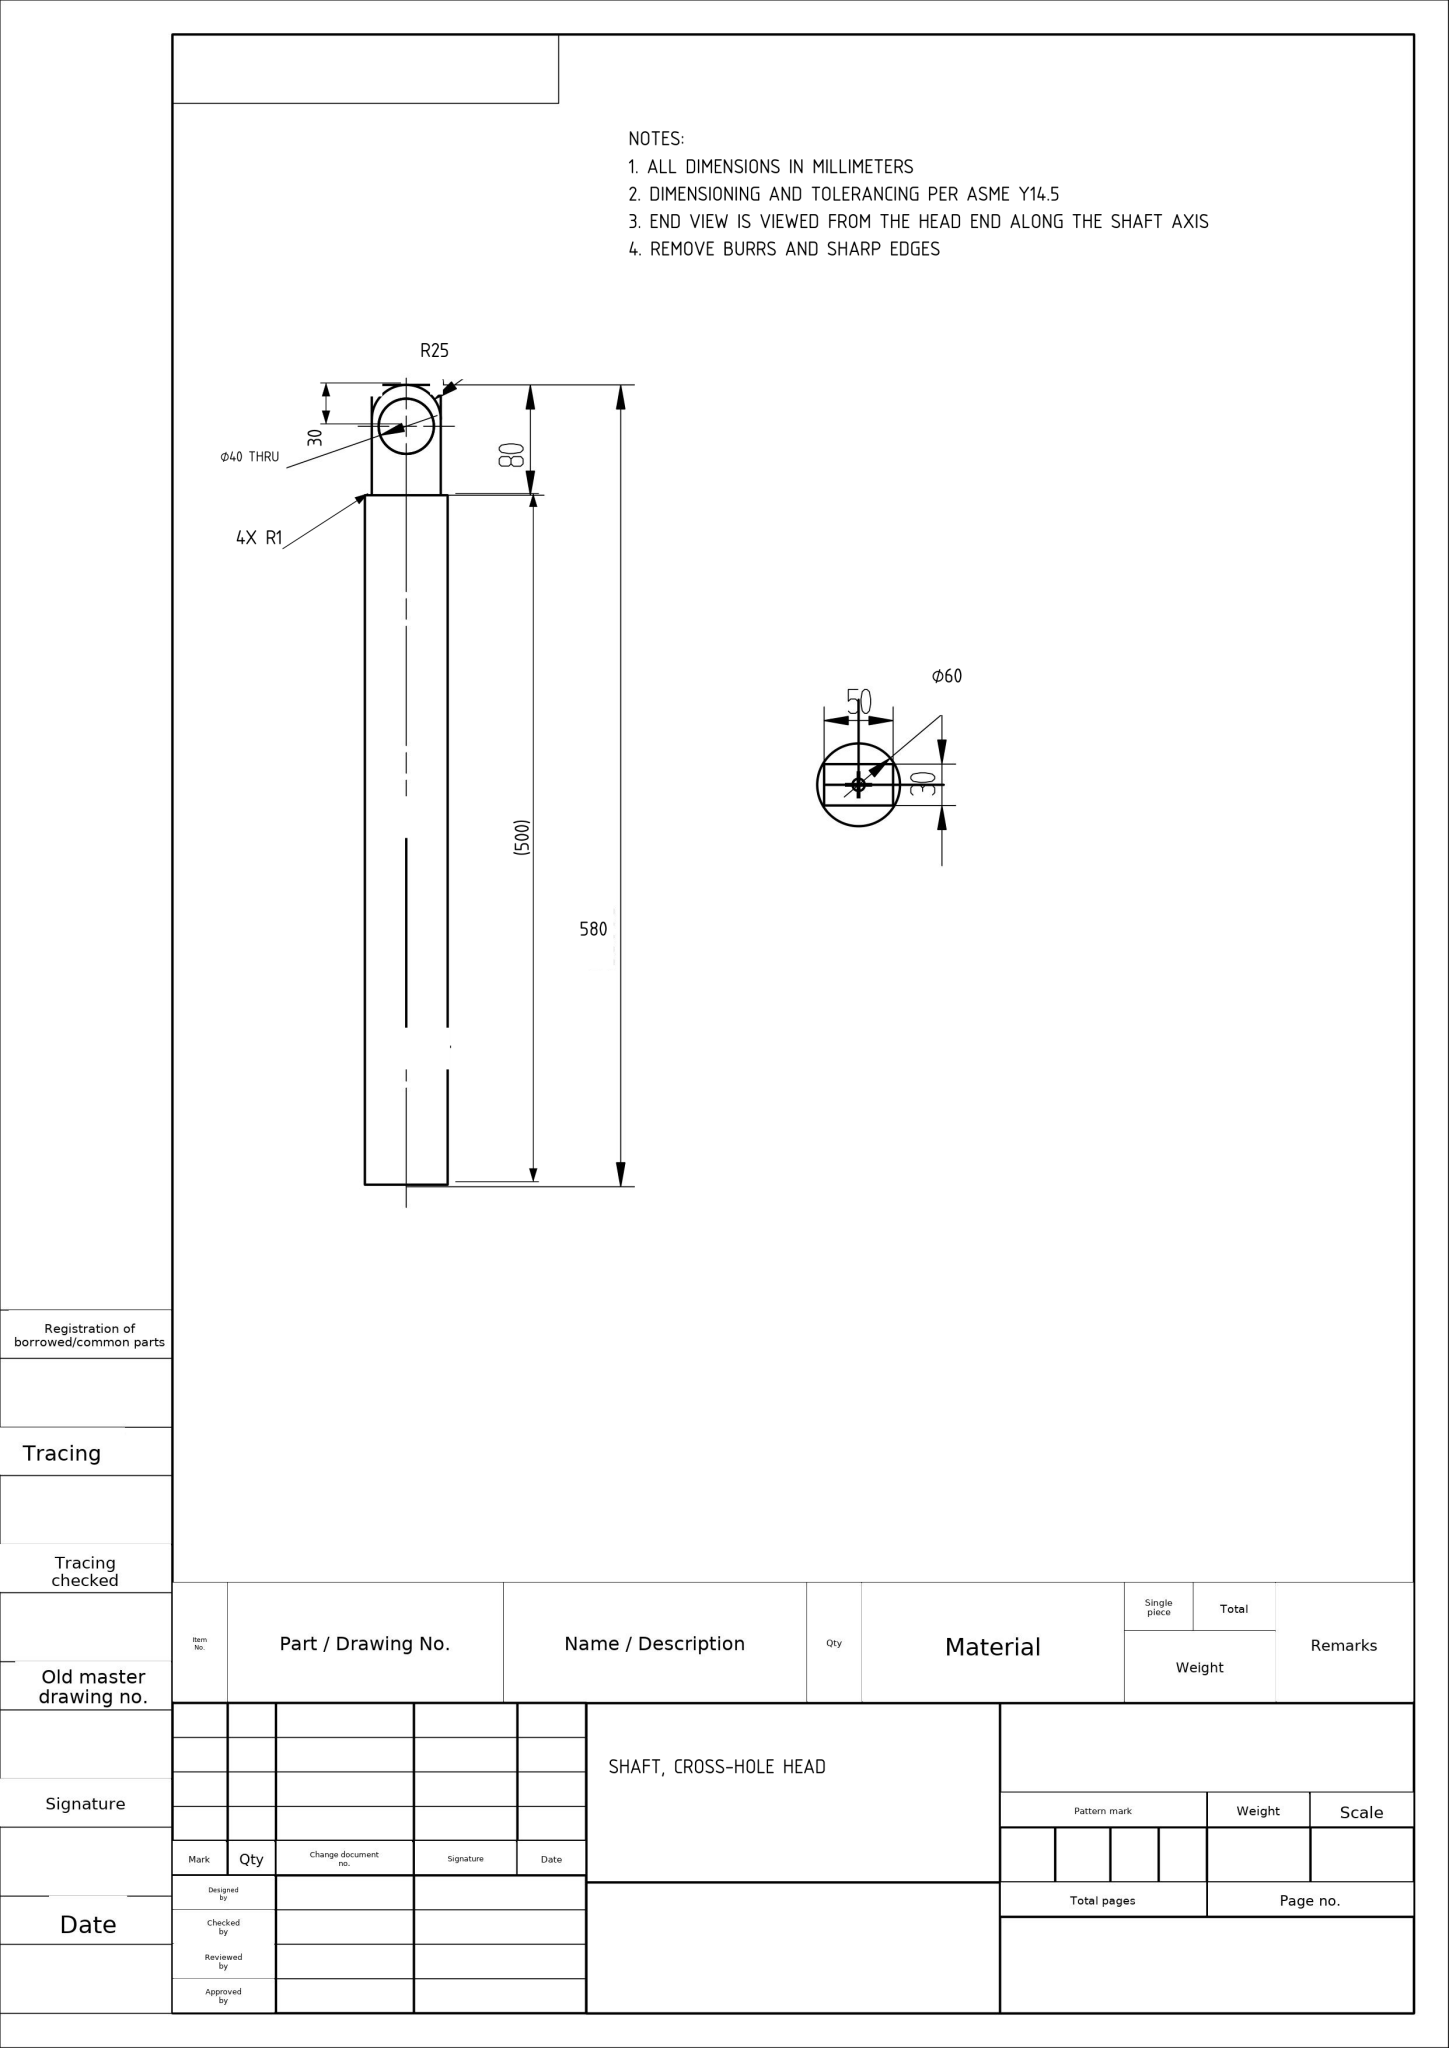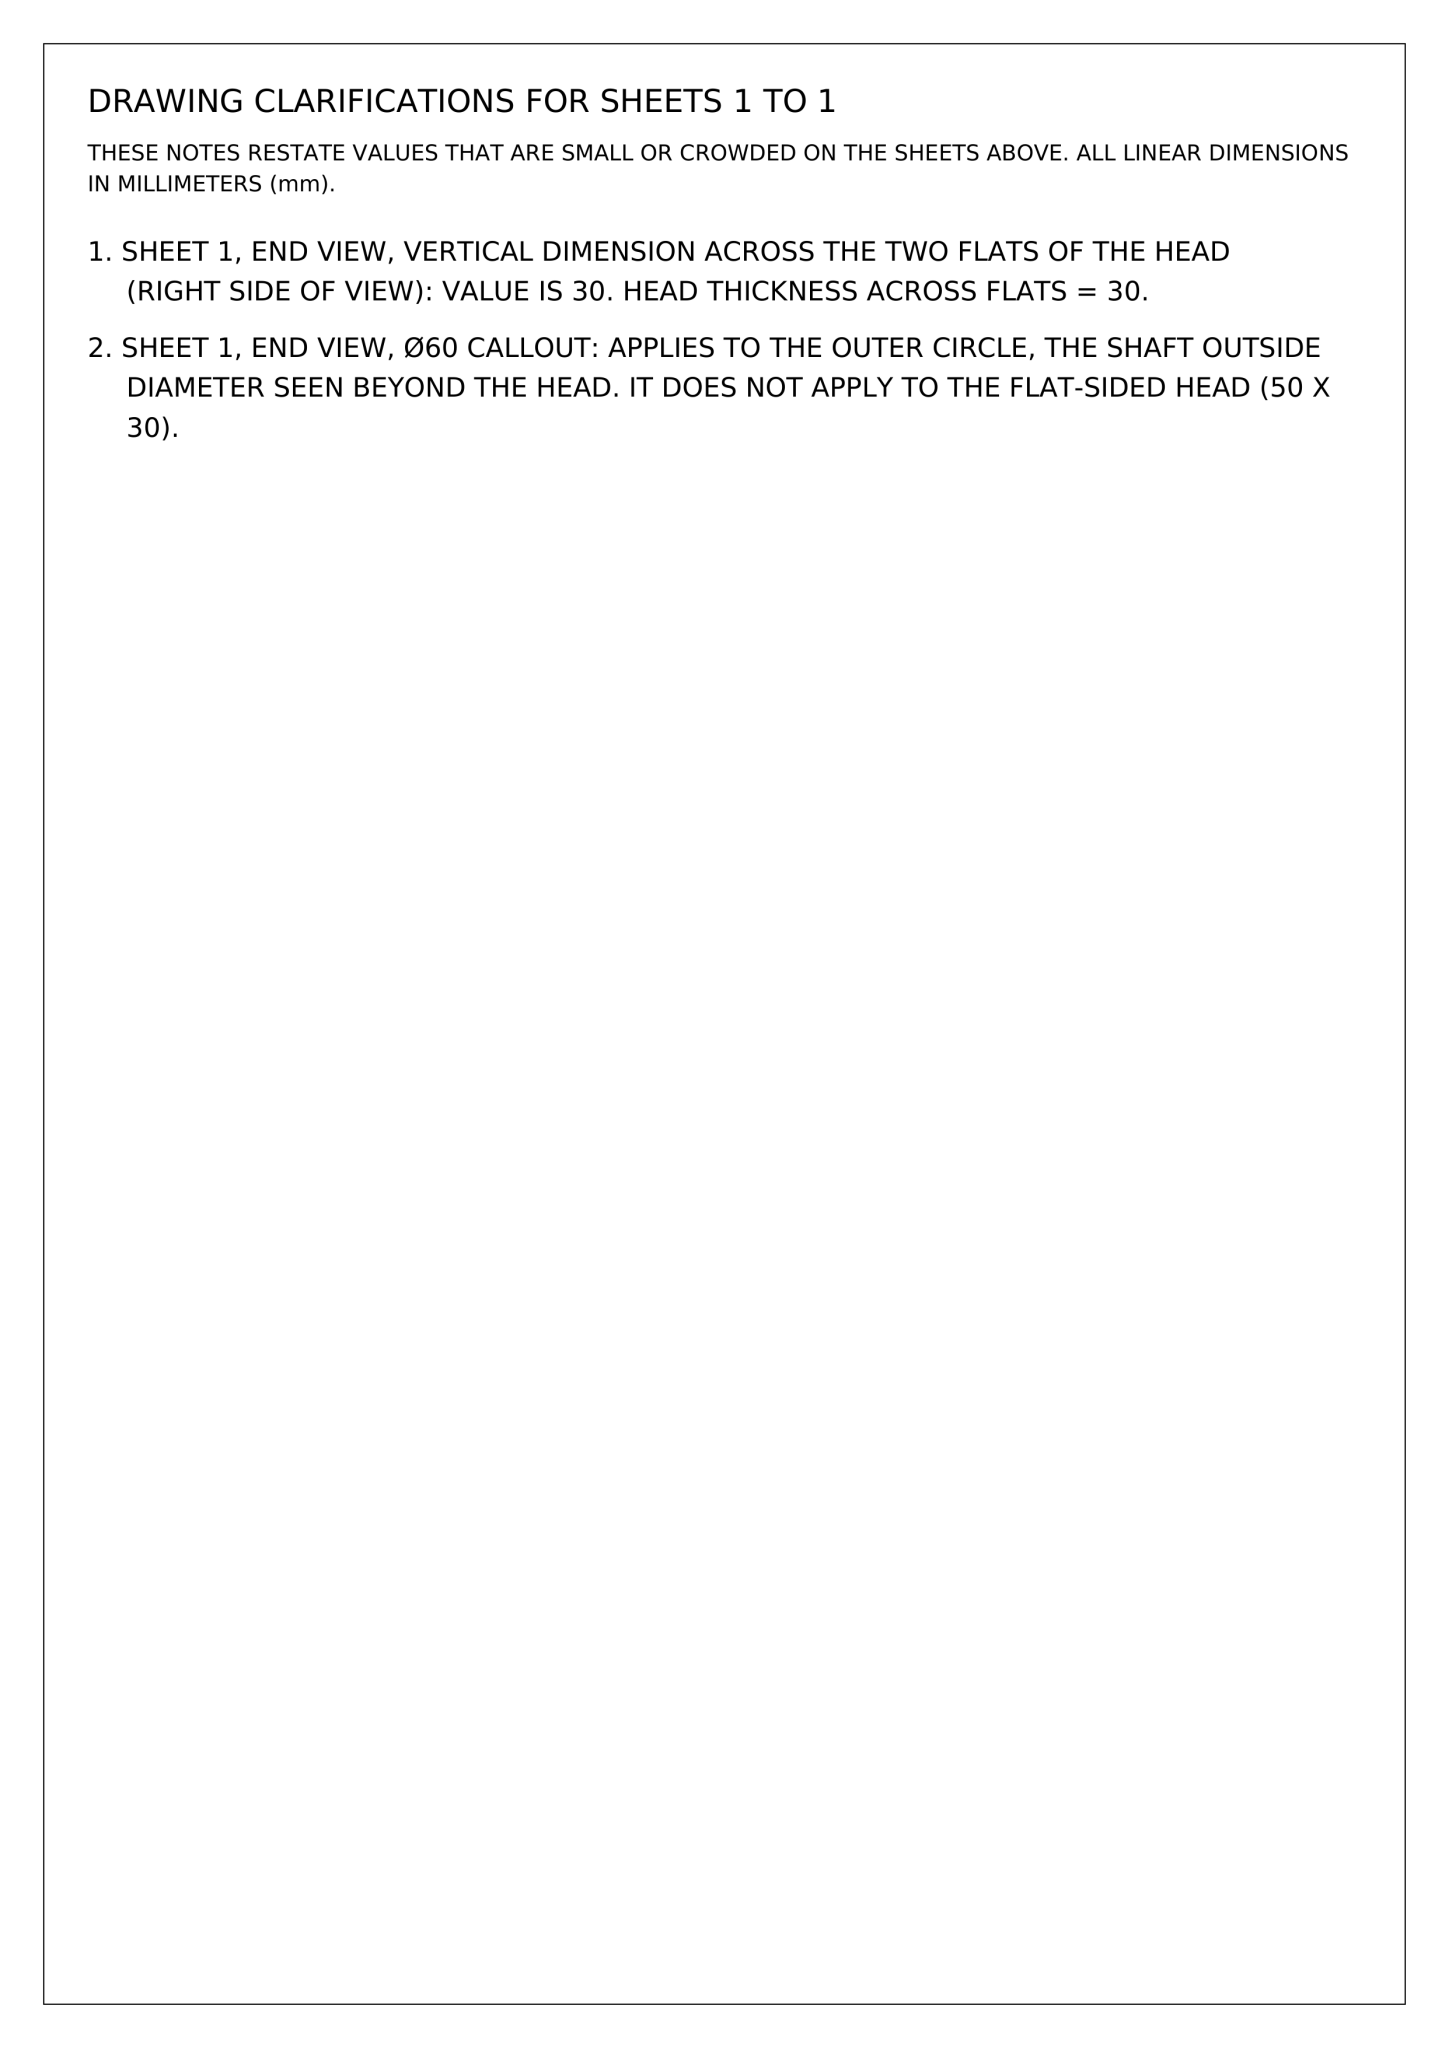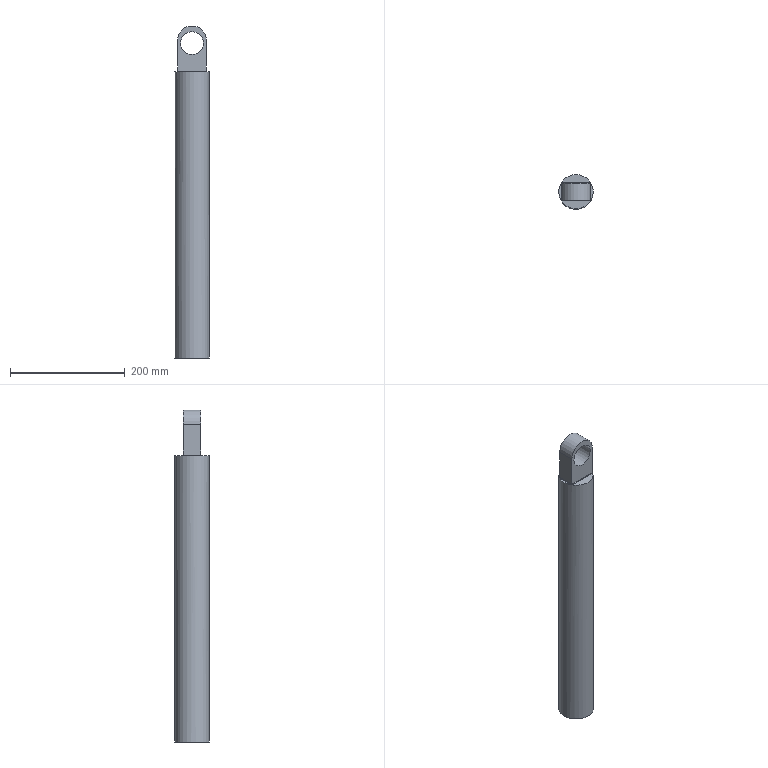Part | NX | mm | 1 solid | 18 faces | box 60 x 60 x 580 mm | volume 1488005 mm3 | plane 9 | cylinder 7 | spline 2 | commonest cylinder face diameters 2 x4 60 x1 40 x1 50 x1
STEP:
#1=CARTESIAN_POINT('',(0.,0.,0.));
#2=DIRECTION('',(0.,0.,1.));
#3=DIRECTION('',(1.,0.,0.));
#4=AXIS2_PLACEMENT_3D('',#1,#2,#3);
#5=(LENGTH_UNIT()NAMED_UNIT(*)SI_UNIT(.MILLI.,.METRE.));
#6=UNCERTAINTY_MEASURE_WITH_UNIT(LENGTH_MEASURE(0.0508),#5,'','');
#7=(NAMED_UNIT(*)PLANE_ANGLE_UNIT()SI_UNIT($,.RADIAN.));
#8=PLANE_ANGLE_MEASURE_WITH_UNIT(PLANE_ANGLE_MEASURE(0.01745),#7);
#9=DIMENSIONAL_EXPONENTS(0.,0.,0.,0.,0.,0.,0.);
#10=(CONVERSION_BASED_UNIT('',#8)NAMED_UNIT(#9)PLANE_ANGLE_UNIT());
#11=(NAMED_UNIT(*)SI_UNIT($,.STERADIAN.)SOLID_ANGLE_UNIT());
#12=(GEOMETRIC_REPRESENTATION_CONTEXT(3)GLOBAL_UNCERTAINTY_ASSIGNED_CONTEXT((#6))GLOBAL_UNIT_ASSIGNED_CONTEXT((#5,#10,#11))REPRESENTATION_CONTEXT('',''));
#13=SHAPE_REPRESENTATION('',(#4),#12);
#14=CARTESIAN_POINT('',(25.377,16.,400.));
#15=VERTEX_POINT('',#14);
#16=CARTESIAN_POINT('',(-25.377,16.,400.));
#17=VERTEX_POINT('',#16);
#18=CARTESIAN_POINT('',(0.,0.,400.));
#19=DIRECTION('',(0.,0.,1.));
#20=DIRECTION('',(1.,0.,0.));
#21=AXIS2_PLACEMENT_3D('',#18,#19,#20);
#22=CIRCLE('',#21,30.);
#23=EDGE_CURVE('',#15,#17,#22,.T.);
#24=ORIENTED_EDGE('',*,*,#23,.T.);
#25=CARTESIAN_POINT('',(0.,16.,400.));
#26=DIRECTION('',(1.,0.,0.));
#27=VECTOR('',#26,1.);
#28=LINE('',#25,#27);
#29=EDGE_CURVE('',#17,#15,#28,.T.);
#30=ORIENTED_EDGE('',*,*,#29,.T.);
#31=EDGE_LOOP('',(#24,#30));
#32=FACE_OUTER_BOUND('',#31,.T.);
#33=CARTESIAN_POINT('',(0.,0.,400.));
#34=DIRECTION('',(0.,0.,1.));
#35=DIRECTION('',(1.,0.,0.));
#36=AXIS2_PLACEMENT_3D('',#33,#34,#35);
#37=PLANE('',#36);
#38=ADVANCED_FACE('',(#32),#37,.T.);
#39=CARTESIAN_POINT('',(-26.,14.967,400.));
#40=VERTEX_POINT('',#39);
#41=CARTESIAN_POINT('',(-26.,-14.967,400.));
#42=VERTEX_POINT('',#41);
#43=CARTESIAN_POINT('',(0.,0.,400.));
#44=DIRECTION('',(0.,0.,1.));
#45=DIRECTION('',(1.,0.,0.));
#46=AXIS2_PLACEMENT_3D('',#43,#44,#45);
#47=CIRCLE('',#46,30.);
#48=EDGE_CURVE('',#40,#42,#47,.T.);
#49=ORIENTED_EDGE('',*,*,#48,.T.);
#50=CARTESIAN_POINT('',(-26.,0.,400.));
#51=DIRECTION('',(0.,1.,0.));
#52=VECTOR('',#51,1.);
#53=LINE('',#50,#52);
#54=EDGE_CURVE('',#42,#40,#53,.T.);
#55=ORIENTED_EDGE('',*,*,#54,.T.);
#56=EDGE_LOOP('',(#49,#55));
#57=FACE_OUTER_BOUND('',#56,.T.);
#58=CARTESIAN_POINT('',(0.,0.,400.));
#59=DIRECTION('',(0.,0.,1.));
#60=DIRECTION('',(1.,0.,0.));
#61=AXIS2_PLACEMENT_3D('',#58,#59,#60);
#62=PLANE('',#61);
#63=ADVANCED_FACE('',(#57),#62,.T.);
#64=CARTESIAN_POINT('',(26.,-14.967,400.));
#65=VERTEX_POINT('',#64);
#66=CARTESIAN_POINT('',(26.,14.967,400.));
#67=VERTEX_POINT('',#66);
#68=CARTESIAN_POINT('',(0.,0.,400.));
#69=DIRECTION('',(0.,0.,1.));
#70=DIRECTION('',(1.,0.,0.));
#71=AXIS2_PLACEMENT_3D('',#68,#69,#70);
#72=CIRCLE('',#71,30.);
#73=EDGE_CURVE('',#65,#67,#72,.T.);
#74=ORIENTED_EDGE('',*,*,#73,.T.);
#75=CARTESIAN_POINT('',(26.,0.,400.));
#76=DIRECTION('',(0.,-1.,0.));
#77=VECTOR('',#76,1.);
#78=LINE('',#75,#77);
#79=EDGE_CURVE('',#67,#65,#78,.T.);
#80=ORIENTED_EDGE('',*,*,#79,.T.);
#81=EDGE_LOOP('',(#74,#80));
#82=FACE_OUTER_BOUND('',#81,.T.);
#83=CARTESIAN_POINT('',(0.,0.,400.));
#84=DIRECTION('',(0.,0.,1.));
#85=DIRECTION('',(1.,0.,0.));
#86=AXIS2_PLACEMENT_3D('',#83,#84,#85);
#87=PLANE('',#86);
#88=ADVANCED_FACE('',(#82),#87,.T.);
#89=CARTESIAN_POINT('',(-25.377,-16.,400.));
#90=VERTEX_POINT('',#89);
#91=CARTESIAN_POINT('',(25.377,-16.,400.));
#92=VERTEX_POINT('',#91);
#93=CARTESIAN_POINT('',(0.,0.,400.));
#94=DIRECTION('',(0.,0.,1.));
#95=DIRECTION('',(1.,0.,0.));
#96=AXIS2_PLACEMENT_3D('',#93,#94,#95);
#97=CIRCLE('',#96,30.);
#98=EDGE_CURVE('',#90,#92,#97,.T.);
#99=ORIENTED_EDGE('',*,*,#98,.T.);
#100=CARTESIAN_POINT('',(-25.,-16.,400.));
#101=DIRECTION('',(-1.,0.,0.));
#102=VECTOR('',#101,1.);
#103=LINE('',#100,#102);
#104=EDGE_CURVE('',#92,#90,#103,.T.);
#105=ORIENTED_EDGE('',*,*,#104,.T.);
#106=EDGE_LOOP('',(#99,#105));
#107=FACE_OUTER_BOUND('',#106,.T.);
#108=CARTESIAN_POINT('',(0.,0.,400.));
#109=DIRECTION('',(0.,0.,1.));
#110=DIRECTION('',(1.,0.,0.));
#111=AXIS2_PLACEMENT_3D('',#108,#109,#110);
#112=PLANE('',#111);
#113=ADVANCED_FACE('',(#107),#112,.T.);
#114=CARTESIAN_POINT('',(25.616,15.616,400.077));
#115=VERTEX_POINT('',#114);
#116=CARTESIAN_POINT('',(25.377,16.,400.));
#117=CARTESIAN_POINT('',(25.459,15.871,400.));
#118=CARTESIAN_POINT('',(25.541,15.739,400.026));
#119=CARTESIAN_POINT('',(25.616,15.616,400.077));
#120=B_SPLINE_CURVE_WITH_KNOTS('',3,(#116,#117,#118,#119),.UNSPECIFIED.,.F.,.F.,(4,4),(0.,1.),.UNSPECIFIED.);
#121=EDGE_CURVE('',#15,#115,#120,.T.);
#122=ORIENTED_EDGE('',*,*,#121,.T.);
#123=CARTESIAN_POINT('',(26.,14.967,400.));
#124=CARTESIAN_POINT('',(25.874,15.186,400.));
#125=CARTESIAN_POINT('',(25.744,15.405,400.023));
#126=CARTESIAN_POINT('',(25.616,15.616,400.077));
#127=B_SPLINE_CURVE_WITH_KNOTS('',3,(#123,#124,#125,#126),.UNSPECIFIED.,.F.,.F.,(4,4),(0.,1.),.UNSPECIFIED.);
#128=EDGE_CURVE('',#67,#115,#127,.T.);
#129=ORIENTED_EDGE('',*,*,#128,.F.);
#130=ORIENTED_EDGE('',*,*,#73,.F.);
#131=CARTESIAN_POINT('',(25.377,-16.,400.));
#132=CARTESIAN_POINT('',(25.379,-15.998,400.));
#133=CARTESIAN_POINT('',(25.38,-15.996,400.));
#134=CARTESIAN_POINT('',(25.419,-15.934,400.));
#135=CARTESIAN_POINT('',(25.458,-15.871,400.));
#136=CARTESIAN_POINT('',(25.539,-15.741,400.));
#137=CARTESIAN_POINT('',(25.58,-15.674,400.));
#138=CARTESIAN_POINT('',(25.663,-15.538,400.));
#139=CARTESIAN_POINT('',(25.705,-15.469,400.));
#140=CARTESIAN_POINT('',(25.83,-15.259,400.));
#141=CARTESIAN_POINT('',(25.915,-15.114,400.));
#142=CARTESIAN_POINT('',(26.,-14.967,400.));
#143=(BOUNDED_CURVE()B_SPLINE_CURVE(3,(#131,#132,#133,#134,#135,#136,#137,#138,#139,#140,#141,#142),.UNSPECIFIED.,.F.,.F.)B_SPLINE_CURVE_WITH_KNOTS((4,2,2,2,2,4),(0.,0.00739,0.2059,0.4044,0.603,1.),.UNSPECIFIED.)CURVE()GEOMETRIC_REPRESENTATION_ITEM()RATIONAL_B_SPLINE_CURVE((1.,1.,1.,1.,1.,1.,1.,1.,1.,1.,1.,1.))REPRESENTATION_ITEM(''));
#144=EDGE_CURVE('',#92,#65,#143,.T.);
#145=ORIENTED_EDGE('',*,*,#144,.F.);
#146=ORIENTED_EDGE('',*,*,#98,.F.);
#147=CARTESIAN_POINT('',(-26.,-14.967,400.));
#148=CARTESIAN_POINT('',(-25.915,-15.114,400.));
#149=CARTESIAN_POINT('',(-25.83,-15.259,400.));
#150=CARTESIAN_POINT('',(-25.705,-15.469,400.));
#151=CARTESIAN_POINT('',(-25.663,-15.538,400.));
#152=CARTESIAN_POINT('',(-25.58,-15.674,400.));
#153=CARTESIAN_POINT('',(-25.539,-15.741,400.));
#154=CARTESIAN_POINT('',(-25.458,-15.871,400.));
#155=CARTESIAN_POINT('',(-25.419,-15.934,400.));
#156=CARTESIAN_POINT('',(-25.38,-15.996,400.));
#157=CARTESIAN_POINT('',(-25.379,-15.998,400.));
#158=CARTESIAN_POINT('',(-25.377,-16.,400.));
#159=(BOUNDED_CURVE()B_SPLINE_CURVE(3,(#147,#148,#149,#150,#151,#152,#153,#154,#155,#156,#157,#158),.UNSPECIFIED.,.F.,.F.)B_SPLINE_CURVE_WITH_KNOTS((4,2,2,2,2,4),(0.,0.397,0.5956,0.7941,0.9926,1.),.UNSPECIFIED.)CURVE()GEOMETRIC_REPRESENTATION_ITEM()RATIONAL_B_SPLINE_CURVE((1.,1.,1.,1.,1.,1.,1.,1.,1.,1.,1.,1.))REPRESENTATION_ITEM(''));
#160=EDGE_CURVE('',#42,#90,#159,.T.);
#161=ORIENTED_EDGE('',*,*,#160,.F.);
#162=ORIENTED_EDGE('',*,*,#48,.F.);
#163=CARTESIAN_POINT('',(-25.616,15.616,400.077));
#164=VERTEX_POINT('',#163);
#165=CARTESIAN_POINT('',(-25.616,15.616,400.077));
#166=CARTESIAN_POINT('',(-25.744,15.405,400.023));
#167=CARTESIAN_POINT('',(-25.874,15.186,400.));
#168=CARTESIAN_POINT('',(-26.,14.967,400.));
#169=B_SPLINE_CURVE_WITH_KNOTS('',3,(#165,#166,#167,#168),.UNSPECIFIED.,.F.,.F.,(4,4),(0.,1.),.UNSPECIFIED.);
#170=EDGE_CURVE('',#164,#40,#169,.T.);
#171=ORIENTED_EDGE('',*,*,#170,.F.);
#172=CARTESIAN_POINT('',(-25.616,15.616,400.077));
#173=CARTESIAN_POINT('',(-25.541,15.739,400.026));
#174=CARTESIAN_POINT('',(-25.459,15.871,400.));
#175=CARTESIAN_POINT('',(-25.377,16.,400.));
#176=B_SPLINE_CURVE_WITH_KNOTS('',3,(#172,#173,#174,#175),.UNSPECIFIED.,.F.,.F.,(4,4),(0.,1.),.UNSPECIFIED.);
#177=EDGE_CURVE('',#164,#17,#176,.T.);
#178=ORIENTED_EDGE('',*,*,#177,.T.);
#179=ORIENTED_EDGE('',*,*,#23,.F.);
#180=EDGE_LOOP('',(#122,#129,#130,#145,#146,#161,#162,#171,#178,#179));
#181=FACE_BOUND('',#180,.T.);
#182=CARTESIAN_POINT('',(30.,0.,-100.));
#183=VERTEX_POINT('',#182);
#184=CARTESIAN_POINT('',(0.,0.,-100.));
#185=DIRECTION('',(0.,0.,1.));
#186=DIRECTION('',(1.,0.,0.));
#187=AXIS2_PLACEMENT_3D('',#184,#185,#186);
#188=CIRCLE('',#187,30.);
#189=EDGE_CURVE('',#183,#183,#188,.T.);
#190=ORIENTED_EDGE('',*,*,#189,.T.);
#191=EDGE_LOOP('',(#190));
#192=FACE_BOUND('',#191,.T.);
#193=CARTESIAN_POINT('',(0.,0.,400.));
#194=DIRECTION('',(0.,0.,-1.));
#195=DIRECTION('',(-1.,0.,0.));
#196=AXIS2_PLACEMENT_3D('',#193,#194,#195);
#197=CYLINDRICAL_SURFACE('',#196,30.);
#198=ADVANCED_FACE('',(#181,#192),#197,.T.);
#199=ORIENTED_EDGE('',*,*,#189,.F.);
#200=EDGE_LOOP('',(#199));
#201=FACE_OUTER_BOUND('',#200,.T.);
#202=CARTESIAN_POINT('',(0.,0.,-100.));
#203=DIRECTION('',(0.,0.,1.));
#204=DIRECTION('',(1.,0.,0.));
#205=AXIS2_PLACEMENT_3D('',#202,#203,#204);
#206=PLANE('',#205);
#207=ADVANCED_FACE('',(#201),#206,.F.);
#208=CARTESIAN_POINT('',(25.,-15.,401.));
#209=VERTEX_POINT('',#208);
#210=CARTESIAN_POINT('',(25.,-15.,455.));
#211=VERTEX_POINT('',#210);
#212=CARTESIAN_POINT('',(25.,-15.,400.));
#213=DIRECTION('',(0.,0.,1.));
#214=VECTOR('',#213,1.);
#215=LINE('',#212,#214);
#216=EDGE_CURVE('',#209,#211,#215,.T.);
#217=ORIENTED_EDGE('',*,*,#216,.F.);
#218=CARTESIAN_POINT('',(25.,-14.967,401.));
#219=VERTEX_POINT('',#218);
#220=CARTESIAN_POINT('',(25.,-15.,401.));
#221=CARTESIAN_POINT('',(25.,-14.989,401.));
#222=CARTESIAN_POINT('',(25.,-14.978,401.));
#223=CARTESIAN_POINT('',(25.,-14.967,401.));
#224=B_SPLINE_CURVE_WITH_KNOTS('',3,(#220,#221,#222,#223),.UNSPECIFIED.,.F.,.F.,(4,4),(0.,1.),.UNSPECIFIED.);
#225=EDGE_CURVE('',#209,#219,#224,.T.);
#226=ORIENTED_EDGE('',*,*,#225,.T.);
#227=CARTESIAN_POINT('',(25.,15.,401.));
#228=VERTEX_POINT('',#227);
#229=CARTESIAN_POINT('',(25.,-15.,401.));
#230=DIRECTION('',(0.,1.,0.));
#231=VECTOR('',#230,1.);
#232=LINE('',#229,#231);
#233=EDGE_CURVE('',#219,#228,#232,.T.);
#234=ORIENTED_EDGE('',*,*,#233,.T.);
#235=CARTESIAN_POINT('',(25.,15.,455.));
#236=VERTEX_POINT('',#235);
#237=CARTESIAN_POINT('',(25.,15.,400.));
#238=DIRECTION('',(0.,0.,1.));
#239=VECTOR('',#238,1.);
#240=LINE('',#237,#239);
#241=EDGE_CURVE('',#228,#236,#240,.T.);
#242=ORIENTED_EDGE('',*,*,#241,.T.);
#243=CARTESIAN_POINT('',(25.,-15.,455.));
#244=DIRECTION('',(0.,-1.,0.));
#245=VECTOR('',#244,1.);
#246=LINE('',#243,#245);
#247=EDGE_CURVE('',#236,#211,#246,.T.);
#248=ORIENTED_EDGE('',*,*,#247,.T.);
#249=EDGE_LOOP('',(#217,#226,#234,#242,#248));
#250=FACE_OUTER_BOUND('',#249,.T.);
#251=CARTESIAN_POINT('',(25.,-15.,400.));
#252=DIRECTION('',(-1.,0.,0.));
#253=DIRECTION('',(0.,0.,1.));
#254=AXIS2_PLACEMENT_3D('',#251,#252,#253);
#255=PLANE('',#254);
#256=ADVANCED_FACE('',(#250),#255,.F.);
#257=CARTESIAN_POINT('',(-25.,15.,455.));
#258=VERTEX_POINT('',#257);
#259=CARTESIAN_POINT('',(-25.,15.,401.));
#260=VERTEX_POINT('',#259);
#261=CARTESIAN_POINT('',(-25.,15.,480.));
#262=DIRECTION('',(-0.,0.,-1.));
#263=VECTOR('',#262,1.);
#264=LINE('',#261,#263);
#265=EDGE_CURVE('',#258,#260,#264,.T.);
#266=ORIENTED_EDGE('',*,*,#265,.T.);
#267=CARTESIAN_POINT('',(-25.,-14.967,401.));
#268=VERTEX_POINT('',#267);
#269=CARTESIAN_POINT('',(-25.,-15.,401.));
#270=DIRECTION('',(0.,-1.,0.));
#271=VECTOR('',#270,1.);
#272=LINE('',#269,#271);
#273=EDGE_CURVE('',#260,#268,#272,.T.);
#274=ORIENTED_EDGE('',*,*,#273,.T.);
#275=CARTESIAN_POINT('',(-25.,-15.,401.));
#276=VERTEX_POINT('',#275);
#277=CARTESIAN_POINT('',(-25.,-14.967,401.));
#278=CARTESIAN_POINT('',(-25.,-14.978,401.));
#279=CARTESIAN_POINT('',(-25.,-14.989,401.));
#280=CARTESIAN_POINT('',(-25.,-15.,401.));
#281=B_SPLINE_CURVE_WITH_KNOTS('',3,(#277,#278,#279,#280),.UNSPECIFIED.,.F.,.F.,(4,4),(0.,1.),.UNSPECIFIED.);
#282=EDGE_CURVE('',#268,#276,#281,.T.);
#283=ORIENTED_EDGE('',*,*,#282,.T.);
#284=CARTESIAN_POINT('',(-25.,-15.,455.));
#285=VERTEX_POINT('',#284);
#286=CARTESIAN_POINT('',(-25.,-15.,480.));
#287=DIRECTION('',(-0.,0.,-1.));
#288=VECTOR('',#287,1.);
#289=LINE('',#286,#288);
#290=EDGE_CURVE('',#285,#276,#289,.T.);
#291=ORIENTED_EDGE('',*,*,#290,.F.);
#292=CARTESIAN_POINT('',(-25.,-15.,455.));
#293=DIRECTION('',(0.,1.,0.));
#294=VECTOR('',#293,1.);
#295=LINE('',#292,#294);
#296=EDGE_CURVE('',#285,#258,#295,.T.);
#297=ORIENTED_EDGE('',*,*,#296,.T.);
#298=EDGE_LOOP('',(#266,#274,#283,#291,#297));
#299=FACE_OUTER_BOUND('',#298,.T.);
#300=CARTESIAN_POINT('',(-25.,-15.,480.));
#301=DIRECTION('',(1.,0.,-0.));
#302=DIRECTION('',(-0.,0.,-1.));
#303=AXIS2_PLACEMENT_3D('',#300,#301,#302);
#304=PLANE('',#303);
#305=ADVANCED_FACE('',(#299),#304,.F.);
#306=CARTESIAN_POINT('',(20.,-15.,450.));
#307=VERTEX_POINT('',#306);
#308=CARTESIAN_POINT('',(0.,-15.,450.));
#309=DIRECTION('',(0.,-1.,0.));
#310=DIRECTION('',(1.,0.,0.));
#311=AXIS2_PLACEMENT_3D('',#308,#309,#310);
#312=CIRCLE('',#311,20.);
#313=EDGE_CURVE('',#307,#307,#312,.T.);
#314=ORIENTED_EDGE('',*,*,#313,.T.);
#315=EDGE_LOOP('',(#314));
#316=FACE_BOUND('',#315,.T.);
#317=CARTESIAN_POINT('',(20.,15.,450.));
#318=VERTEX_POINT('',#317);
#319=CARTESIAN_POINT('',(0.,15.,450.));
#320=DIRECTION('',(0.,-1.,0.));
#321=DIRECTION('',(1.,0.,0.));
#322=AXIS2_PLACEMENT_3D('',#319,#320,#321);
#323=CIRCLE('',#322,20.);
#324=EDGE_CURVE('',#318,#318,#323,.T.);
#325=ORIENTED_EDGE('',*,*,#324,.F.);
#326=EDGE_LOOP('',(#325));
#327=FACE_BOUND('',#326,.T.);
#328=CARTESIAN_POINT('',(0.,-15.,450.));
#329=DIRECTION('',(0.,1.,0.));
#330=DIRECTION('',(0.,0.,1.));
#331=AXIS2_PLACEMENT_3D('',#328,#329,#330);
#332=CYLINDRICAL_SURFACE('',#331,20.);
#333=ADVANCED_FACE('',(#316,#327),#332,.F.);
#334=ORIENTED_EDGE('',*,*,#290,.T.);
#335=CARTESIAN_POINT('',(25.,-15.,401.));
#336=DIRECTION('',(1.,0.,0.));
#337=VECTOR('',#336,1.);
#338=LINE('',#335,#337);
#339=EDGE_CURVE('',#276,#209,#338,.T.);
#340=ORIENTED_EDGE('',*,*,#339,.T.);
#341=ORIENTED_EDGE('',*,*,#216,.T.);
#342=CARTESIAN_POINT('',(0.,-15.,455.));
#343=DIRECTION('',(0.,-1.,0.));
#344=DIRECTION('',(0.,0.,-1.));
#345=AXIS2_PLACEMENT_3D('',#342,#343,#344);
#346=CIRCLE('',#345,25.);
#347=EDGE_CURVE('',#211,#285,#346,.T.);
#348=ORIENTED_EDGE('',*,*,#347,.T.);
#349=EDGE_LOOP('',(#334,#340,#341,#348));
#350=FACE_BOUND('',#349,.T.);
#351=ORIENTED_EDGE('',*,*,#313,.F.);
#352=EDGE_LOOP('',(#351));
#353=FACE_BOUND('',#352,.T.);
#354=CARTESIAN_POINT('',(0.,-15.,450.));
#355=DIRECTION('',(0.,-1.,0.));
#356=DIRECTION('',(0.,0.,-1.));
#357=AXIS2_PLACEMENT_3D('',#354,#355,#356);
#358=PLANE('',#357);
#359=ADVANCED_FACE('',(#350,#353),#358,.T.);
#360=ORIENTED_EDGE('',*,*,#241,.F.);
#361=CARTESIAN_POINT('',(0.,15.,401.));
#362=DIRECTION('',(-1.,0.,0.));
#363=VECTOR('',#362,1.);
#364=LINE('',#361,#363);
#365=EDGE_CURVE('',#228,#260,#364,.T.);
#366=ORIENTED_EDGE('',*,*,#365,.T.);
#367=ORIENTED_EDGE('',*,*,#265,.F.);
#368=CARTESIAN_POINT('',(0.,15.,455.));
#369=DIRECTION('',(0.,1.,0.));
#370=DIRECTION('',(0.,0.,-1.));
#371=AXIS2_PLACEMENT_3D('',#368,#369,#370);
#372=CIRCLE('',#371,25.);
#373=EDGE_CURVE('',#258,#236,#372,.T.);
#374=ORIENTED_EDGE('',*,*,#373,.T.);
#375=EDGE_LOOP('',(#360,#366,#367,#374));
#376=FACE_BOUND('',#375,.T.);
#377=ORIENTED_EDGE('',*,*,#324,.T.);
#378=EDGE_LOOP('',(#377));
#379=FACE_BOUND('',#378,.T.);
#380=CARTESIAN_POINT('',(0.,15.,450.));
#381=DIRECTION('',(0.,-1.,0.));
#382=DIRECTION('',(0.,0.,-1.));
#383=AXIS2_PLACEMENT_3D('',#380,#381,#382);
#384=PLANE('',#383);
#385=ADVANCED_FACE('',(#376,#379),#384,.F.);
#386=ORIENTED_EDGE('',*,*,#373,.F.);
#387=ORIENTED_EDGE('',*,*,#296,.F.);
#388=ORIENTED_EDGE('',*,*,#347,.F.);
#389=ORIENTED_EDGE('',*,*,#247,.F.);
#390=EDGE_LOOP('',(#386,#387,#388,#389));
#391=FACE_OUTER_BOUND('',#390,.T.);
#392=CARTESIAN_POINT('',(0.,-15.,455.));
#393=DIRECTION('',(0.,1.,0.));
#394=DIRECTION('',(0.,0.,1.));
#395=AXIS2_PLACEMENT_3D('',#392,#393,#394);
#396=CYLINDRICAL_SURFACE('',#395,25.);
#397=ADVANCED_FACE('',(#391),#396,.T.);
#398=CARTESIAN_POINT('',(25.,-15.,401.));
#399=CARTESIAN_POINT('',(25.,-15.,400.715));
#400=CARTESIAN_POINT('',(25.125,-15.114,400.47));
#401=CARTESIAN_POINT('',(25.357,-15.387,400.2));
#402=CARTESIAN_POINT('',(25.43,-15.467,400.14));
#403=CARTESIAN_POINT('',(25.508,-15.75,400.02));
#404=CARTESIAN_POINT('',(25.458,-15.872,400.));
#405=CARTESIAN_POINT('',(25.377,-16.,400.));
#406=B_SPLINE_CURVE_WITH_KNOTS('',3,(#398,#399,#400,#401,#402,#403,#404,#405),.UNSPECIFIED.,.F.,.F.,(4,2,2,4),(0.,0.5,0.75,1.),.UNSPECIFIED.);
#407=EDGE_CURVE('',#209,#92,#406,.T.);
#408=ORIENTED_EDGE('',*,*,#407,.F.);
#409=ORIENTED_EDGE('',*,*,#339,.F.);
#410=CARTESIAN_POINT('',(-25.377,-16.,400.));
#411=CARTESIAN_POINT('',(-25.539,-15.743,400.));
#412=CARTESIAN_POINT('',(-25.433,-15.478,400.11));
#413=CARTESIAN_POINT('',(-25.126,-15.115,400.469));
#414=CARTESIAN_POINT('',(-25.,-15.,400.714));
#415=CARTESIAN_POINT('',(-25.,-15.,401.));
#416=B_SPLINE_CURVE_WITH_KNOTS('',3,(#410,#411,#412,#413,#414,#415),.UNSPECIFIED.,.F.,.F.,(4,2,4),(0.,0.5,1.),.UNSPECIFIED.);
#417=EDGE_CURVE('',#90,#276,#416,.T.);
#418=ORIENTED_EDGE('',*,*,#417,.F.);
#419=ORIENTED_EDGE('',*,*,#104,.F.);
#420=EDGE_LOOP('',(#408,#409,#418,#419));
#421=FACE_OUTER_BOUND('',#420,.T.);
#422=CARTESIAN_POINT('',(0.,-16.,401.));
#423=DIRECTION('',(-1.,0.,0.));
#424=DIRECTION('',(0.,0.,1.));
#425=AXIS2_PLACEMENT_3D('',#422,#423,#424);
#426=CYLINDRICAL_SURFACE('',#425,1.);
#427=ADVANCED_FACE('',(#421),#426,.F.);
#428=ORIENTED_EDGE('',*,*,#417,.T.);
#429=ORIENTED_EDGE('',*,*,#282,.F.);
#430=CARTESIAN_POINT('',(-26.,-14.967,400.));
#431=CARTESIAN_POINT('',(-25.476,-14.967,400.));
#432=CARTESIAN_POINT('',(-25.,-14.967,400.476));
#433=CARTESIAN_POINT('',(-25.,-14.967,401.));
#434=B_SPLINE_CURVE_WITH_KNOTS('',3,(#430,#431,#432,#433),.UNSPECIFIED.,.F.,.F.,(4,4),(0.,1.),.UNSPECIFIED.);
#435=EDGE_CURVE('',#42,#268,#434,.T.);
#436=ORIENTED_EDGE('',*,*,#435,.F.);
#437=ORIENTED_EDGE('',*,*,#160,.T.);
#438=EDGE_LOOP('',(#428,#429,#436,#437));
#439=FACE_OUTER_BOUND('',#438,.T.);
#440=CARTESIAN_POINT('',(-25.,-14.967,401.));
#441=CARTESIAN_POINT('',(-25.,-15.163,401.));
#442=CARTESIAN_POINT('',(-25.,-15.358,400.986));
#443=CARTESIAN_POINT('',(-25.,-15.646,400.94));
#444=CARTESIAN_POINT('',(-25.,-15.742,400.921));
#445=CARTESIAN_POINT('',(-25.,-15.931,400.872));
#446=CARTESIAN_POINT('',(-25.,-16.025,400.843));
#447=CARTESIAN_POINT('',(-25.,-16.209,400.772));
#448=CARTESIAN_POINT('',(-25.,-16.298,400.731));
#449=CARTESIAN_POINT('',(-25.,-16.469,400.633));
#450=CARTESIAN_POINT('',(-25.,-16.549,400.577));
#451=CARTESIAN_POINT('',(-25.,-16.658,400.479));
#452=CARTESIAN_POINT('',(-25.,-16.692,400.444));
#453=CARTESIAN_POINT('',(-25.,-16.754,400.368));
#454=CARTESIAN_POINT('',(-25.,-16.783,400.327));
#455=CARTESIAN_POINT('',(-25.,-16.853,400.197));
#456=CARTESIAN_POINT('',(-25.,-16.882,400.099));
#457=CARTESIAN_POINT('',(-25.,-16.882,400.));
#458=CARTESIAN_POINT('',(-25.,-14.967,400.));
#459=CARTESIAN_POINT('',(-25.,-15.108,400.082));
#460=CARTESIAN_POINT('',(-25.,-15.265,400.147));
#461=CARTESIAN_POINT('',(-25.,-15.507,400.215));
#462=CARTESIAN_POINT('',(-25.,-15.588,400.233));
#463=CARTESIAN_POINT('',(-25.,-15.748,400.259));
#464=CARTESIAN_POINT('',(-25.,-15.829,400.267));
#465=CARTESIAN_POINT('',(-25.,-15.988,400.272));
#466=CARTESIAN_POINT('',(-25.,-16.066,400.27));
#467=CARTESIAN_POINT('',(-25.,-16.217,400.252));
#468=CARTESIAN_POINT('',(-25.,-16.288,400.237));
#469=CARTESIAN_POINT('',(-25.,-16.385,400.204));
#470=CARTESIAN_POINT('',(-25.,-16.415,400.191));
#471=CARTESIAN_POINT('',(-25.,-16.471,400.162));
#472=CARTESIAN_POINT('',(-25.,-16.497,400.145));
#473=CARTESIAN_POINT('',(-25.,-16.56,400.09));
#474=CARTESIAN_POINT('',(-25.,-16.586,400.045));
#475=CARTESIAN_POINT('',(-25.,-16.586,400.));
#476=CARTESIAN_POINT('',(-26.,-14.967,400.));
#477=CARTESIAN_POINT('',(-25.915,-15.114,400.));
#478=CARTESIAN_POINT('',(-25.83,-15.259,400.));
#479=CARTESIAN_POINT('',(-25.705,-15.469,400.));
#480=CARTESIAN_POINT('',(-25.663,-15.538,400.));
#481=CARTESIAN_POINT('',(-25.58,-15.674,400.));
#482=CARTESIAN_POINT('',(-25.539,-15.741,400.));
#483=CARTESIAN_POINT('',(-25.458,-15.871,400.));
#484=CARTESIAN_POINT('',(-25.419,-15.934,400.));
#485=CARTESIAN_POINT('',(-25.344,-16.053,400.));
#486=CARTESIAN_POINT('',(-25.308,-16.109,400.));
#487=CARTESIAN_POINT('',(-25.26,-16.184,400.));
#488=CARTESIAN_POINT('',(-25.245,-16.207,400.));
#489=CARTESIAN_POINT('',(-25.218,-16.25,400.));
#490=CARTESIAN_POINT('',(-25.205,-16.27,400.));
#491=CARTESIAN_POINT('',(-25.174,-16.318,400.));
#492=CARTESIAN_POINT('',(-25.161,-16.338,400.));
#493=CARTESIAN_POINT('',(-25.161,-16.337,400.));
#494=(BOUNDED_SURFACE()B_SPLINE_SURFACE(2,3,((#440,#441,#442,#443,#444,#445,#446,#447,#448,#449,#450,#451,#452,#453,#454,#455,#456,#457),(#458,#459,#460,#461,#462,#463,#464,#465,#466,#467,#468,#469,#470,#471,#472,#473,#474,#475),(#476,#477,#478,#479,#480,#481,#482,#483,#484,#485,#486,#487,#488,#489,#490,#491,#492,#493)),.UNSPECIFIED.,.F.,.F.,.F.)B_SPLINE_SURFACE_WITH_KNOTS((3,3),(4,2,2,2,2,2,2,2,4),(0.,1.),(0.,0.25,0.375,0.5,0.625,0.75,0.8125,0.875,1.),.UNSPECIFIED.)GEOMETRIC_REPRESENTATION_ITEM()RATIONAL_B_SPLINE_SURFACE(((1.,1.,1.,1.,1.,1.,1.,1.,1.,1.,1.,1.,1.,1.,1.,1.,1.,1.),(0.7071,0.7371,0.7652,0.8049,0.8178,0.8427,0.8549,0.8781,0.8892,0.9101,0.9198,0.9326,0.9367,0.944,0.9473,0.9556,0.9589,0.9588),(1.,1.,1.,1.,1.,1.,1.,1.,1.,1.,1.,1.,1.,1.,1.,1.,1.,1.)))REPRESENTATION_ITEM('')SURFACE());
#495=ADVANCED_FACE('',(#439),#494,.T.);
#496=ORIENTED_EDGE('',*,*,#407,.T.);
#497=ORIENTED_EDGE('',*,*,#144,.T.);
#498=CARTESIAN_POINT('',(25.,-14.967,401.));
#499=CARTESIAN_POINT('',(25.,-14.967,400.476));
#500=CARTESIAN_POINT('',(25.476,-14.967,400.));
#501=CARTESIAN_POINT('',(26.,-14.967,400.));
#502=B_SPLINE_CURVE_WITH_KNOTS('',3,(#498,#499,#500,#501),.UNSPECIFIED.,.F.,.F.,(4,4),(0.,1.),.UNSPECIFIED.);
#503=EDGE_CURVE('',#219,#65,#502,.T.);
#504=ORIENTED_EDGE('',*,*,#503,.F.);
#505=ORIENTED_EDGE('',*,*,#225,.F.);
#506=EDGE_LOOP('',(#496,#497,#504,#505));
#507=FACE_OUTER_BOUND('',#506,.T.);
#508=CARTESIAN_POINT('',(26.,-14.967,400.));
#509=CARTESIAN_POINT('',(25.915,-15.114,400.));
#510=CARTESIAN_POINT('',(25.83,-15.259,400.));
#511=CARTESIAN_POINT('',(25.705,-15.469,400.));
#512=CARTESIAN_POINT('',(25.663,-15.538,400.));
#513=CARTESIAN_POINT('',(25.58,-15.674,400.));
#514=CARTESIAN_POINT('',(25.539,-15.741,400.));
#515=CARTESIAN_POINT('',(25.458,-15.871,400.));
#516=CARTESIAN_POINT('',(25.419,-15.934,400.));
#517=CARTESIAN_POINT('',(25.344,-16.053,400.));
#518=CARTESIAN_POINT('',(25.308,-16.109,400.));
#519=CARTESIAN_POINT('',(25.26,-16.184,400.));
#520=CARTESIAN_POINT('',(25.245,-16.207,400.));
#521=CARTESIAN_POINT('',(25.218,-16.25,400.));
#522=CARTESIAN_POINT('',(25.205,-16.27,400.));
#523=CARTESIAN_POINT('',(25.174,-16.318,400.));
#524=CARTESIAN_POINT('',(25.161,-16.338,400.));
#525=CARTESIAN_POINT('',(25.161,-16.337,400.));
#526=CARTESIAN_POINT('',(25.,-14.967,400.));
#527=CARTESIAN_POINT('',(25.,-15.108,400.082));
#528=CARTESIAN_POINT('',(25.,-15.265,400.147));
#529=CARTESIAN_POINT('',(25.,-15.507,400.215));
#530=CARTESIAN_POINT('',(25.,-15.588,400.233));
#531=CARTESIAN_POINT('',(25.,-15.748,400.259));
#532=CARTESIAN_POINT('',(25.,-15.829,400.267));
#533=CARTESIAN_POINT('',(25.,-15.988,400.272));
#534=CARTESIAN_POINT('',(25.,-16.066,400.27));
#535=CARTESIAN_POINT('',(25.,-16.217,400.252));
#536=CARTESIAN_POINT('',(25.,-16.288,400.237));
#537=CARTESIAN_POINT('',(25.,-16.385,400.204));
#538=CARTESIAN_POINT('',(25.,-16.415,400.191));
#539=CARTESIAN_POINT('',(25.,-16.471,400.162));
#540=CARTESIAN_POINT('',(25.,-16.497,400.145));
#541=CARTESIAN_POINT('',(25.,-16.56,400.09));
#542=CARTESIAN_POINT('',(25.,-16.586,400.045));
#543=CARTESIAN_POINT('',(25.,-16.586,400.));
#544=CARTESIAN_POINT('',(25.,-14.967,401.));
#545=CARTESIAN_POINT('',(25.,-15.163,401.));
#546=CARTESIAN_POINT('',(25.,-15.358,400.986));
#547=CARTESIAN_POINT('',(25.,-15.646,400.94));
#548=CARTESIAN_POINT('',(25.,-15.742,400.921));
#549=CARTESIAN_POINT('',(25.,-15.931,400.872));
#550=CARTESIAN_POINT('',(25.,-16.025,400.843));
#551=CARTESIAN_POINT('',(25.,-16.209,400.772));
#552=CARTESIAN_POINT('',(25.,-16.298,400.731));
#553=CARTESIAN_POINT('',(25.,-16.469,400.633));
#554=CARTESIAN_POINT('',(25.,-16.549,400.577));
#555=CARTESIAN_POINT('',(25.,-16.658,400.479));
#556=CARTESIAN_POINT('',(25.,-16.692,400.444));
#557=CARTESIAN_POINT('',(25.,-16.754,400.368));
#558=CARTESIAN_POINT('',(25.,-16.783,400.327));
#559=CARTESIAN_POINT('',(25.,-16.853,400.197));
#560=CARTESIAN_POINT('',(25.,-16.882,400.099));
#561=CARTESIAN_POINT('',(25.,-16.882,400.));
#562=(BOUNDED_SURFACE()B_SPLINE_SURFACE(2,3,((#508,#509,#510,#511,#512,#513,#514,#515,#516,#517,#518,#519,#520,#521,#522,#523,#524,#525),(#526,#527,#528,#529,#530,#531,#532,#533,#534,#535,#536,#537,#538,#539,#540,#541,#542,#543),(#544,#545,#546,#547,#548,#549,#550,#551,#552,#553,#554,#555,#556,#557,#558,#559,#560,#561)),.UNSPECIFIED.,.F.,.F.,.F.)B_SPLINE_SURFACE_WITH_KNOTS((3,3),(4,2,2,2,2,2,2,2,4),(0.,1.),(0.,0.25,0.375,0.5,0.625,0.75,0.8125,0.875,1.),.UNSPECIFIED.)GEOMETRIC_REPRESENTATION_ITEM()RATIONAL_B_SPLINE_SURFACE(((1.,1.,1.,1.,1.,1.,1.,1.,1.,1.,1.,1.,1.,1.,1.,1.,1.,1.),(0.7071,0.7371,0.7652,0.8049,0.8178,0.8427,0.8549,0.8781,0.8892,0.9101,0.9198,0.9326,0.9367,0.944,0.9473,0.9556,0.9589,0.9588),(1.,1.,1.,1.,1.,1.,1.,1.,1.,1.,1.,1.,1.,1.,1.,1.,1.,1.)))REPRESENTATION_ITEM('')SURFACE());
#563=ADVANCED_FACE('',(#507),#562,.T.);
#564=ORIENTED_EDGE('',*,*,#435,.T.);
#565=ORIENTED_EDGE('',*,*,#273,.F.);
#566=CARTESIAN_POINT('',(-26.,16.,401.));
#567=DIRECTION('',(-0.7071,-0.7071,0.));
#568=DIRECTION('',(0.7071,-0.7071,0.));
#569=AXIS2_PLACEMENT_3D('',#566,#567,#568);
#570=ELLIPSE('',#569,1.414,1.);
#571=EDGE_CURVE('',#164,#260,#570,.T.);
#572=ORIENTED_EDGE('',*,*,#571,.F.);
#573=ORIENTED_EDGE('',*,*,#170,.T.);
#574=ORIENTED_EDGE('',*,*,#54,.F.);
#575=EDGE_LOOP('',(#564,#565,#572,#573,#574));
#576=FACE_OUTER_BOUND('',#575,.T.);
#577=CARTESIAN_POINT('',(-26.,0.,401.));
#578=DIRECTION('',(0.,1.,0.));
#579=DIRECTION('',(0.,0.,1.));
#580=AXIS2_PLACEMENT_3D('',#577,#578,#579);
#581=CYLINDRICAL_SURFACE('',#580,1.);
#582=ADVANCED_FACE('',(#576),#581,.F.);
#583=ORIENTED_EDGE('',*,*,#79,.F.);
#584=ORIENTED_EDGE('',*,*,#128,.T.);
#585=CARTESIAN_POINT('',(26.,16.,401.));
#586=DIRECTION('',(0.7071,-0.7071,0.));
#587=DIRECTION('',(0.7071,0.7071,0.));
#588=AXIS2_PLACEMENT_3D('',#585,#586,#587);
#589=ELLIPSE('',#588,1.414,1.);
#590=EDGE_CURVE('',#228,#115,#589,.T.);
#591=ORIENTED_EDGE('',*,*,#590,.F.);
#592=ORIENTED_EDGE('',*,*,#233,.F.);
#593=ORIENTED_EDGE('',*,*,#503,.T.);
#594=EDGE_LOOP('',(#583,#584,#591,#592,#593));
#595=FACE_OUTER_BOUND('',#594,.T.);
#596=CARTESIAN_POINT('',(26.,-15.,401.));
#597=DIRECTION('',(0.,1.,0.));
#598=DIRECTION('',(0.,0.,1.));
#599=AXIS2_PLACEMENT_3D('',#596,#597,#598);
#600=CYLINDRICAL_SURFACE('',#599,1.);
#601=ADVANCED_FACE('',(#595),#600,.F.);
#602=ORIENTED_EDGE('',*,*,#571,.T.);
#603=ORIENTED_EDGE('',*,*,#365,.F.);
#604=ORIENTED_EDGE('',*,*,#590,.T.);
#605=ORIENTED_EDGE('',*,*,#121,.F.);
#606=ORIENTED_EDGE('',*,*,#29,.F.);
#607=ORIENTED_EDGE('',*,*,#177,.F.);
#608=EDGE_LOOP('',(#602,#603,#604,#605,#606,#607));
#609=FACE_OUTER_BOUND('',#608,.T.);
#610=CARTESIAN_POINT('',(0.,16.,401.));
#611=DIRECTION('',(1.,0.,0.));
#612=DIRECTION('',(0.,0.,-1.));
#613=AXIS2_PLACEMENT_3D('',#610,#611,#612);
#614=CYLINDRICAL_SURFACE('',#613,1.);
#615=ADVANCED_FACE('',(#609),#614,.F.);
#616=CLOSED_SHELL('',(#38,#63,#88,#113,#198,#207,#256,#305,#333,#359,#385,#397,#427,#495,#563,#582,#601,#615));
#617=MANIFOLD_SOLID_BREP('',#616);
#618=ADVANCED_BREP_SHAPE_REPRESENTATION('',(#617),#12);
#619=SHAPE_REPRESENTATION_RELATIONSHIP('','',#13,#618);
#620=PRESENTATION_LAYER_ASSIGNMENT('','',(#617));
#621=COLOUR_RGB('',1.,0.6,0.);
#622=FILL_AREA_STYLE_COLOUR('',#621);
#623=FILL_AREA_STYLE('',(#622));
#624=SURFACE_STYLE_FILL_AREA(#623);
#625=SURFACE_SIDE_STYLE('',(#624));
#626=SURFACE_STYLE_USAGE(.BOTH.,#625);
#627=PRESENTATION_STYLE_ASSIGNMENT((#626));
#628=STYLED_ITEM('',(#627),#617);
#629=MECHANICAL_DESIGN_GEOMETRIC_PRESENTATION_REPRESENTATION('',(#628),#12);